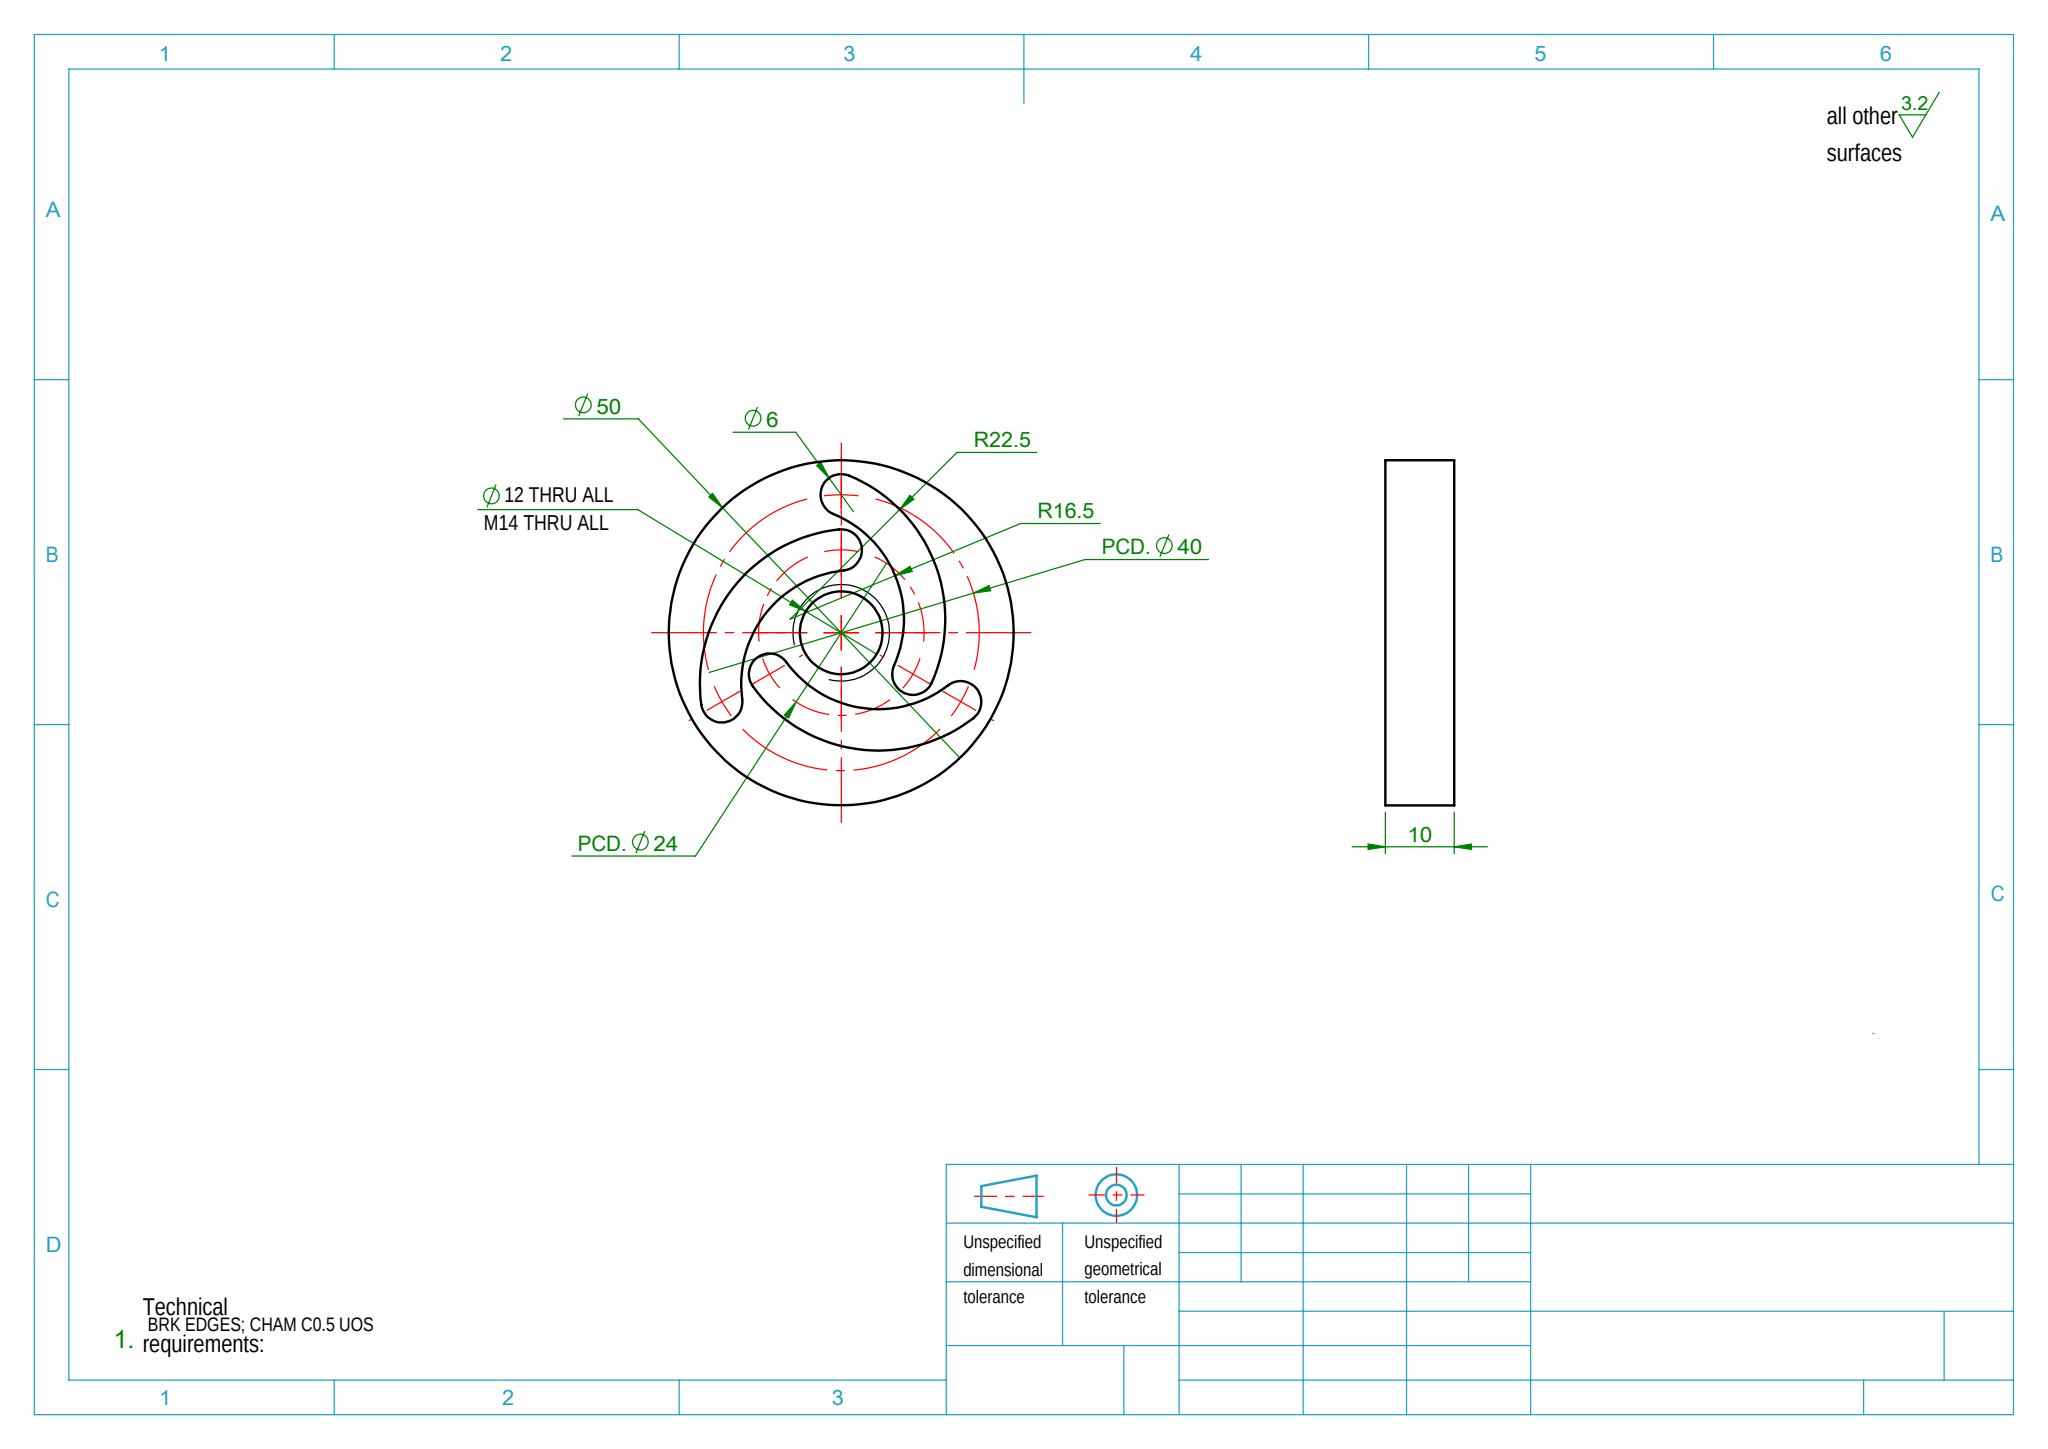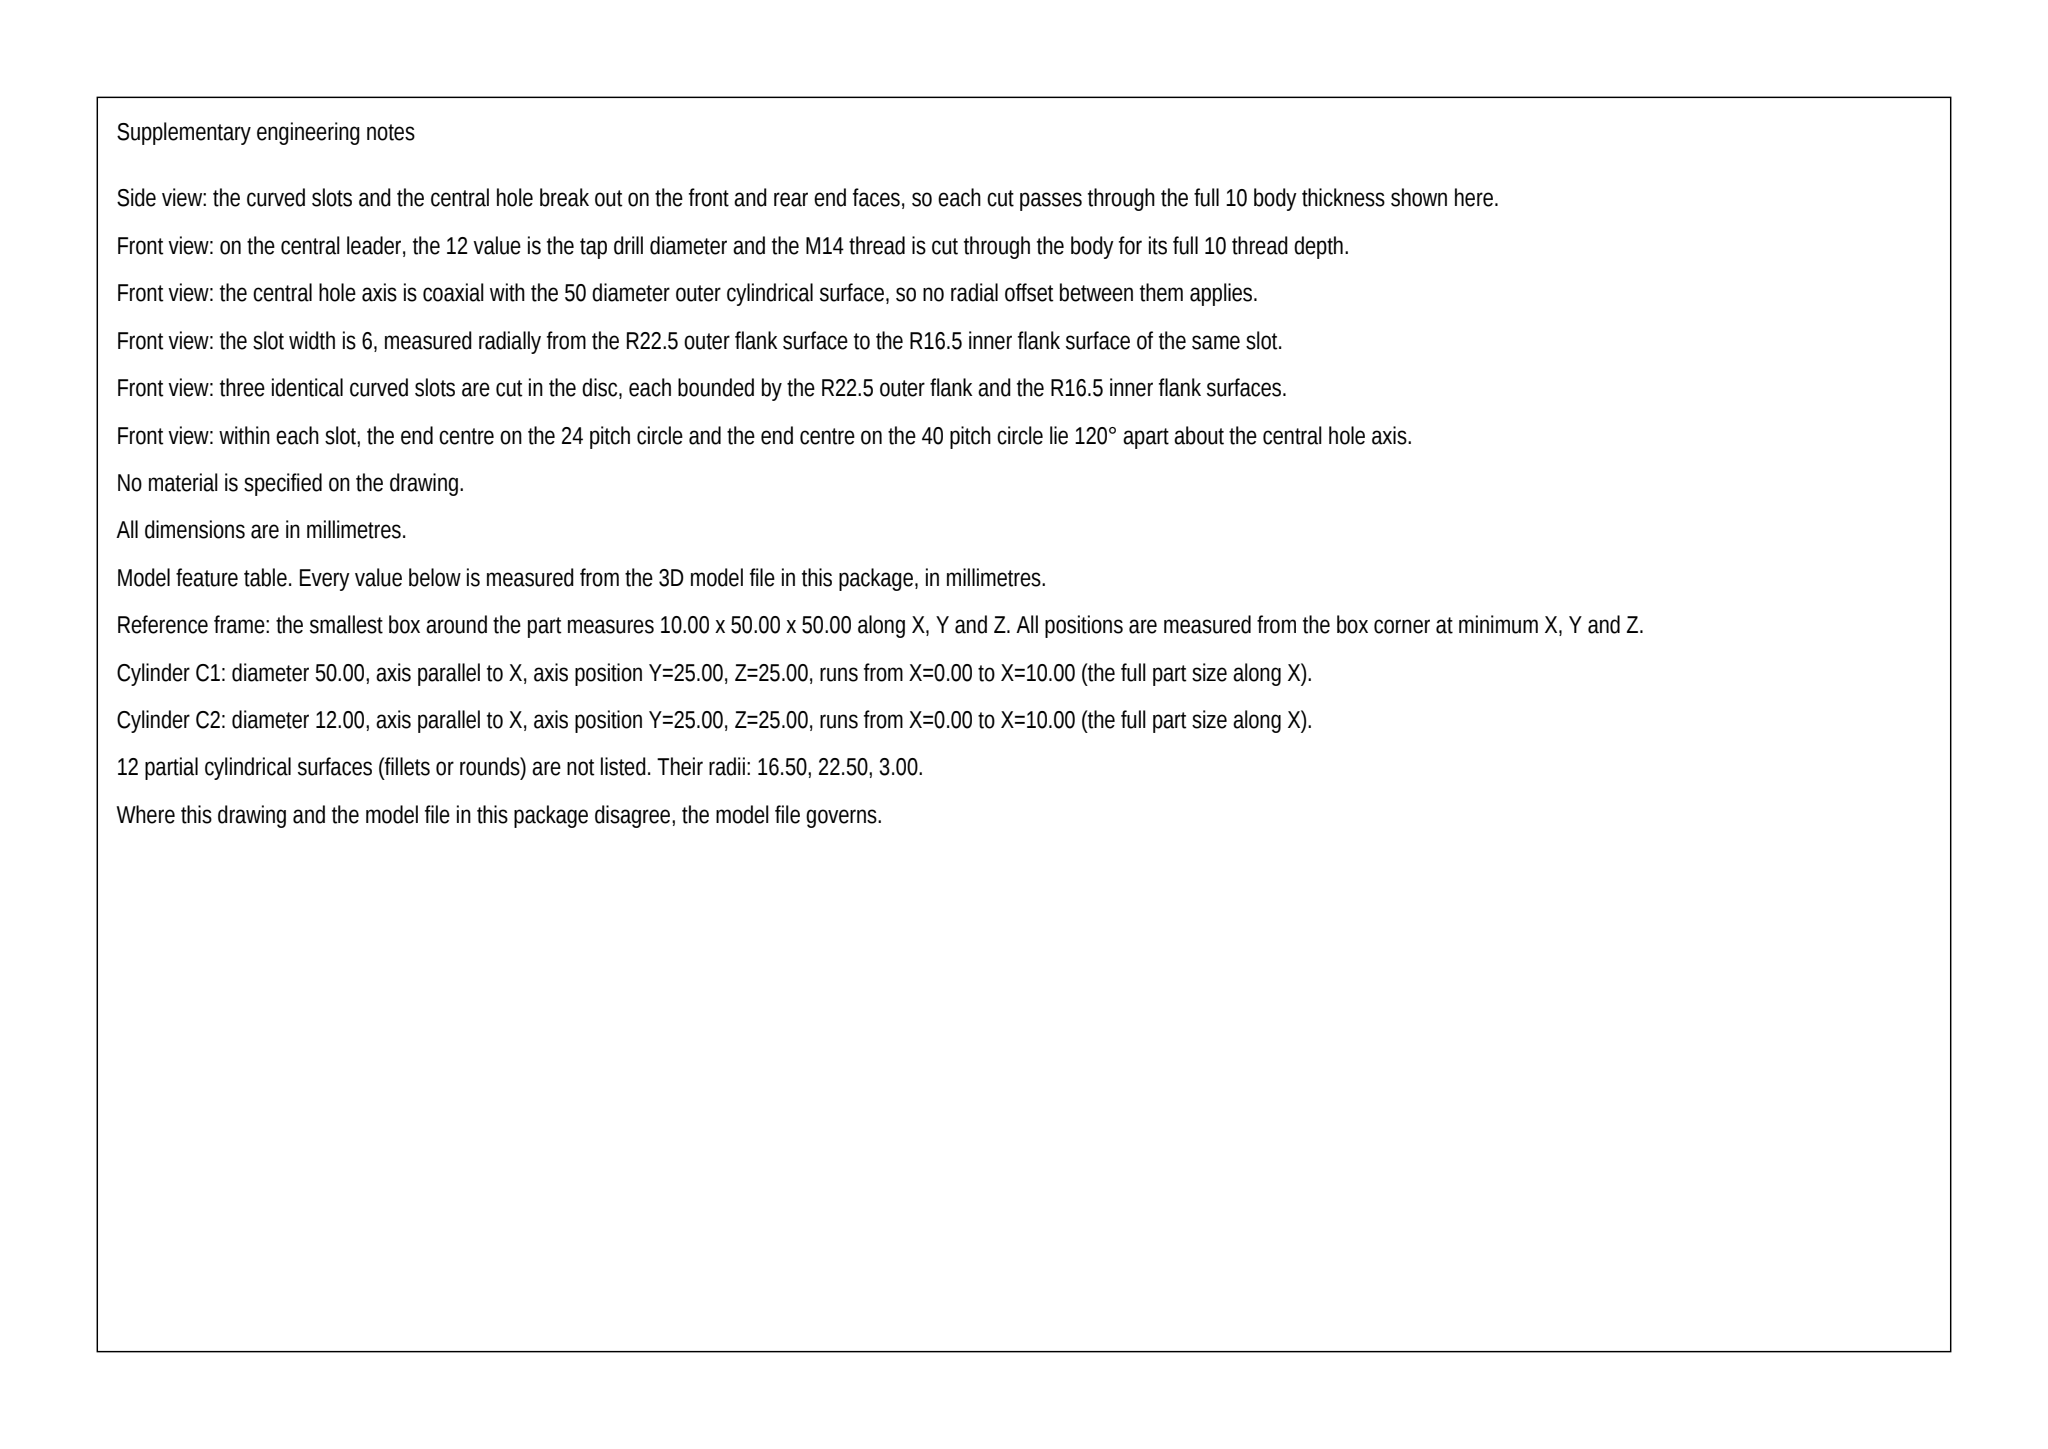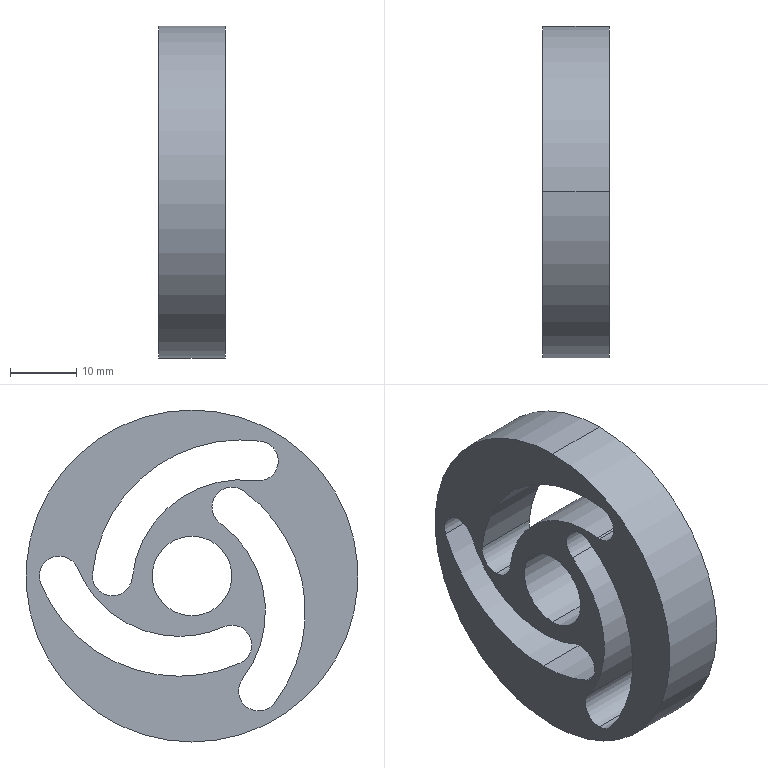Part | SolidWorks | mm | 1 solid | 23 faces | box 10 x 50 x 50 mm | volume 12034 mm3 | cylinder 21 | plane 2 | commonest cylinder face diameters 6 x9 33 x4 45 x4 12 x2 50 x2
Drawing notes:
3X SLOT ARC CTR: 7.67 FROM AXIS, 120° APART, R16.5/R22.5 | from the solid: R16.5/R22.5 arc centres at (17.6,23.0),(26.96,32.41),(30.43,19.6) vs part axis (25,25): offset 7.67, 120° apart
SLOT ENDS Ø6: PCD Ø24 END ON HORIZ CL, PCD Ø40 END 120° CCW | from the solid: Ø6 end-cap axes at r=12 (0°,120°,240°) and r=20 (0°,120°,240°) from axis (25,25); each slot links r=12 end to r=20 end 120° away, mean slot radius R19.5
3X CURVED SLOT THRU ALL (10) | from the solid: All Ø6/R16.5/R22.5 slot cylinders length 10 along x, between faces x=0 and x=10
build123d program:
from build123d import *

# Parameters (mm, degrees)
SKETCH1_R           = 25
BOSS_EXTRUDE1_DEPTH = 10
M14_TAPPED_HOLE1_D  = 12
CUT_EXTRUDE2_DEPTH  = 37.742
CIRPATTERN2_COUNT   = 3


with BuildPart() as part:
    # Sketch1 → Boss-Extrude1 (new body)
    with BuildSketch(Plane(origin=(0, 0, 0), x_dir=(0, 0, -1), z_dir=(1, 0, 0))):
        Circle(SKETCH1_R)
    extrude(amount=BOSS_EXTRUDE1_DEPTH)

    # M14 Tapped Hole1 (through all)
    with Locations(Plane(origin=(10, 0, 0), x_dir=(0, 0, -1), z_dir=(1, 0, 0))):
        with Locations((0, 0)):
            Hole(M14_TAPPED_HOLE1_D / 2)

    # Sketch7 → Cut-Extrude2 (cut, through all)
    with BuildSketch(Plane(origin=(10, 0, 0), x_dir=(0, 0, -1), z_dir=(1, 0, 0))):
        with BuildLine():
            ThreePointArc((-20.294, -10.401), (-16.92, -12.973), (-14.347, -9.599))
            ThreePointArc((-14.347, -9.599), (-10.959, 2.81), (0.3085, 9.016))
            ThreePointArc((0.3085, 9.016), (2.984, 12.308), (-0.3085, 14.984))
            ThreePointArc((-0.3085, 14.984), (-15.674, 6.522), (-20.294, -10.401))
        make_face()
    cut_extrude2 = extrude(amount=-CUT_EXTRUDE2_DEPTH, mode=Mode.SUBTRACT)

    # CirPattern2: Cut-Extrude2 ×3 about axis
    cirpattern2_axis = Axis((0, 0, 0), (1, 0, 0))
    for i in range(1, CIRPATTERN2_COUNT):
        add(cut_extrude2.rotate(cirpattern2_axis, i * 360 / CIRPATTERN2_COUNT), mode=Mode.SUBTRACT)


solid = part.part
STEP:
#1=CARTESIAN_POINT('',(0.,-10.,-20.321));
#2=VERTEX_POINT('',#1);
#3=CARTESIAN_POINT('',(0.,-7.625,-15.487));
#4=VERTEX_POINT('',#3);
#5=CARTESIAN_POINT('',(0.,-10.,-17.321));
#6=DIRECTION('',(1.,0.,0.));
#7=DIRECTION('',(0.,0.866,0.5));
#8=AXIS2_PLACEMENT_3D('',#5,#6,#7);
#9=CIRCLE('',#8,3.);
#10=EDGE_CURVE('',#2,#4,#9,.T.);
#11=ORIENTED_EDGE('',*,*,#10,.F.);
#12=CARTESIAN_POINT('',(10.,-10.,-20.321));
#13=VERTEX_POINT('',#12);
#14=CARTESIAN_POINT('',(0.,-10.,-20.321));
#15=DIRECTION('',(1.,0.,0.));
#16=VECTOR('',#15,1000.);
#17=LINE('',#14,#16);
#18=EDGE_CURVE('',#2,#13,#17,.T.);
#19=ORIENTED_EDGE('',*,*,#18,.T.);
#20=CARTESIAN_POINT('',(10.,-7.625,-15.487));
#21=VERTEX_POINT('',#20);
#22=CARTESIAN_POINT('',(10.,-10.,-17.321));
#23=DIRECTION('',(1.,0.,0.));
#24=DIRECTION('',(0.,0.866,0.5));
#25=AXIS2_PLACEMENT_3D('',#22,#23,#24);
#26=CIRCLE('',#25,3.);
#27=EDGE_CURVE('',#13,#21,#26,.T.);
#28=ORIENTED_EDGE('',*,*,#27,.T.);
#29=CARTESIAN_POINT('',(0.,-7.625,-15.487));
#30=DIRECTION('',(1.,0.,0.));
#31=VECTOR('',#30,1000.);
#32=LINE('',#29,#31);
#33=EDGE_CURVE('',#4,#21,#32,.T.);
#34=ORIENTED_EDGE('',*,*,#33,.F.);
#35=EDGE_LOOP('',(#11,#19,#28,#34));
#36=FACE_OUTER_BOUND('',#35,.T.);
#37=CARTESIAN_POINT('',(0.,-10.,-17.321));
#38=DIRECTION('',(1.,0.,0.));
#39=DIRECTION('',(0.,0.,-1.));
#40=AXIS2_PLACEMENT_3D('',#37,#38,#39);
#41=CYLINDRICAL_SURFACE('',#40,3.);
#42=ADVANCED_FACE('',(#36),#41,.F.);
#43=CARTESIAN_POINT('',(0.,1.962,-9.092));
#44=VERTEX_POINT('',#43);
#45=CARTESIAN_POINT('',(0.,-4.775,-7.654));
#46=VERTEX_POINT('',#45);
#47=CARTESIAN_POINT('',(0.,1.962,7.408));
#48=DIRECTION('',(-1.,0.,0.));
#49=DIRECTION('',(0.,-0.866,0.5));
#50=AXIS2_PLACEMENT_3D('',#47,#48,#49);
#51=CIRCLE('',#50,16.5);
#52=EDGE_CURVE('',#44,#46,#51,.T.);
#53=ORIENTED_EDGE('',*,*,#52,.F.);
#54=CARTESIAN_POINT('',(10.,1.962,-9.092));
#55=VERTEX_POINT('',#54);
#56=CARTESIAN_POINT('',(0.,1.962,-9.092));
#57=DIRECTION('',(1.,0.,0.));
#58=VECTOR('',#57,1000.);
#59=LINE('',#56,#58);
#60=EDGE_CURVE('',#44,#55,#59,.T.);
#61=ORIENTED_EDGE('',*,*,#60,.T.);
#62=CARTESIAN_POINT('',(10.,-4.775,-7.654));
#63=VERTEX_POINT('',#62);
#64=CARTESIAN_POINT('',(10.,1.962,7.408));
#65=DIRECTION('',(-1.,0.,0.));
#66=DIRECTION('',(0.,-0.866,0.5));
#67=AXIS2_PLACEMENT_3D('',#64,#65,#66);
#68=CIRCLE('',#67,16.5);
#69=EDGE_CURVE('',#55,#63,#68,.T.);
#70=ORIENTED_EDGE('',*,*,#69,.T.);
#71=CARTESIAN_POINT('',(0.,-4.775,-7.654));
#72=DIRECTION('',(1.,0.,0.));
#73=VECTOR('',#72,1000.);
#74=LINE('',#71,#73);
#75=EDGE_CURVE('',#46,#63,#74,.T.);
#76=ORIENTED_EDGE('',*,*,#75,.F.);
#77=EDGE_LOOP('',(#53,#61,#70,#76));
#78=FACE_OUTER_BOUND('',#77,.T.);
#79=CARTESIAN_POINT('',(0.,1.962,7.408));
#80=DIRECTION('',(1.,0.,0.));
#81=DIRECTION('',(0.,0.,-1.));
#82=AXIS2_PLACEMENT_3D('',#79,#80,#81);
#83=CYLINDRICAL_SURFACE('',#82,16.5);
#84=ADVANCED_FACE('',(#78),#83,.T.);
#85=CARTESIAN_POINT('',(0.,1.962,-15.092));
#86=VERTEX_POINT('',#85);
#87=CARTESIAN_POINT('',(0.,22.775,-1.14));
#88=VERTEX_POINT('',#87);
#89=CARTESIAN_POINT('',(0.,1.962,7.408));
#90=DIRECTION('',(1.,0.,0.));
#91=DIRECTION('',(0.,-0.866,0.5));
#92=AXIS2_PLACEMENT_3D('',#89,#90,#91);
#93=CIRCLE('',#92,22.5);
#94=EDGE_CURVE('',#86,#88,#93,.T.);
#95=ORIENTED_EDGE('',*,*,#94,.F.);
#96=CARTESIAN_POINT('',(10.,1.962,-15.092));
#97=VERTEX_POINT('',#96);
#98=CARTESIAN_POINT('',(0.,1.962,-15.092));
#99=DIRECTION('',(1.,0.,0.));
#100=VECTOR('',#99,1000.);
#101=LINE('',#98,#100);
#102=EDGE_CURVE('',#86,#97,#101,.T.);
#103=ORIENTED_EDGE('',*,*,#102,.T.);
#104=CARTESIAN_POINT('',(10.,22.775,-1.14));
#105=VERTEX_POINT('',#104);
#106=CARTESIAN_POINT('',(10.,1.962,7.408));
#107=DIRECTION('',(1.,0.,0.));
#108=DIRECTION('',(0.,-0.866,0.5));
#109=AXIS2_PLACEMENT_3D('',#106,#107,#108);
#110=CIRCLE('',#109,22.5);
#111=EDGE_CURVE('',#97,#105,#110,.T.);
#112=ORIENTED_EDGE('',*,*,#111,.T.);
#113=CARTESIAN_POINT('',(0.,22.775,-1.14));
#114=DIRECTION('',(1.,0.,0.));
#115=VECTOR('',#114,1000.);
#116=LINE('',#113,#115);
#117=EDGE_CURVE('',#88,#105,#116,.T.);
#118=ORIENTED_EDGE('',*,*,#117,.F.);
#119=EDGE_LOOP('',(#95,#103,#112,#118));
#120=FACE_OUTER_BOUND('',#119,.T.);
#121=CARTESIAN_POINT('',(0.,1.962,7.408));
#122=DIRECTION('',(1.,0.,0.));
#123=DIRECTION('',(0.,0.,-1.));
#124=AXIS2_PLACEMENT_3D('',#121,#122,#123);
#125=CYLINDRICAL_SURFACE('',#124,22.5);
#126=ADVANCED_FACE('',(#120),#125,.F.);
#127=CARTESIAN_POINT('',(0.,-10.,14.321));
#128=VERTEX_POINT('',#127);
#129=CARTESIAN_POINT('',(0.,-9.599,14.347));
#130=VERTEX_POINT('',#129);
#131=CARTESIAN_POINT('',(0.,-10.,17.321));
#132=DIRECTION('',(1.,0.,0.));
#133=DIRECTION('',(0.,0.,-1.));
#134=AXIS2_PLACEMENT_3D('',#131,#132,#133);
#135=CIRCLE('',#134,3.);
#136=EDGE_CURVE('',#128,#130,#135,.T.);
#137=ORIENTED_EDGE('',*,*,#136,.F.);
#138=CARTESIAN_POINT('',(10.,-10.,14.321));
#139=VERTEX_POINT('',#138);
#140=CARTESIAN_POINT('',(0.,-10.,14.321));
#141=DIRECTION('',(1.,0.,0.));
#142=VECTOR('',#141,1000.);
#143=LINE('',#140,#142);
#144=EDGE_CURVE('',#128,#139,#143,.T.);
#145=ORIENTED_EDGE('',*,*,#144,.T.);
#146=CARTESIAN_POINT('',(10.,-9.599,14.347));
#147=VERTEX_POINT('',#146);
#148=CARTESIAN_POINT('',(10.,-10.,17.321));
#149=DIRECTION('',(1.,0.,0.));
#150=DIRECTION('',(0.,0.,-1.));
#151=AXIS2_PLACEMENT_3D('',#148,#149,#150);
#152=CIRCLE('',#151,3.);
#153=EDGE_CURVE('',#139,#147,#152,.T.);
#154=ORIENTED_EDGE('',*,*,#153,.T.);
#155=CARTESIAN_POINT('',(0.,-9.599,14.347));
#156=DIRECTION('',(1.,0.,0.));
#157=VECTOR('',#156,1000.);
#158=LINE('',#155,#157);
#159=EDGE_CURVE('',#130,#147,#158,.T.);
#160=ORIENTED_EDGE('',*,*,#159,.F.);
#161=EDGE_LOOP('',(#137,#145,#154,#160));
#162=FACE_OUTER_BOUND('',#161,.T.);
#163=CARTESIAN_POINT('',(0.,-10.,17.321));
#164=DIRECTION('',(1.,0.,0.));
#165=DIRECTION('',(0.,0.,-1.));
#166=AXIS2_PLACEMENT_3D('',#163,#164,#165);
#167=CYLINDRICAL_SURFACE('',#166,3.);
#168=ADVANCED_FACE('',(#162),#167,.F.);
#169=CARTESIAN_POINT('',(0.,12.,-3.));
#170=VERTEX_POINT('',#169);
#171=CARTESIAN_POINT('',(0.,14.984,0.3085));
#172=VERTEX_POINT('',#171);
#173=CARTESIAN_POINT('',(0.,12.,0.));
#174=DIRECTION('',(1.,0.,0.));
#175=DIRECTION('',(0.,0.,-1.));
#176=AXIS2_PLACEMENT_3D('',#173,#174,#175);
#177=CIRCLE('',#176,3.);
#178=EDGE_CURVE('',#170,#172,#177,.T.);
#179=ORIENTED_EDGE('',*,*,#178,.F.);
#180=CARTESIAN_POINT('',(10.,12.,-3.));
#181=VERTEX_POINT('',#180);
#182=CARTESIAN_POINT('',(0.,12.,-3.));
#183=DIRECTION('',(1.,0.,0.));
#184=VECTOR('',#183,1000.);
#185=LINE('',#182,#184);
#186=EDGE_CURVE('',#170,#181,#185,.T.);
#187=ORIENTED_EDGE('',*,*,#186,.T.);
#188=CARTESIAN_POINT('',(10.,14.984,0.3085));
#189=VERTEX_POINT('',#188);
#190=CARTESIAN_POINT('',(10.,12.,0.));
#191=DIRECTION('',(1.,0.,0.));
#192=DIRECTION('',(0.,0.,-1.));
#193=AXIS2_PLACEMENT_3D('',#190,#191,#192);
#194=CIRCLE('',#193,3.);
#195=EDGE_CURVE('',#181,#189,#194,.T.);
#196=ORIENTED_EDGE('',*,*,#195,.T.);
#197=CARTESIAN_POINT('',(0.,14.984,0.3085));
#198=DIRECTION('',(1.,0.,0.));
#199=VECTOR('',#198,1000.);
#200=LINE('',#197,#199);
#201=EDGE_CURVE('',#172,#189,#200,.T.);
#202=ORIENTED_EDGE('',*,*,#201,.F.);
#203=EDGE_LOOP('',(#179,#187,#196,#202));
#204=FACE_OUTER_BOUND('',#203,.T.);
#205=CARTESIAN_POINT('',(0.,12.,0.));
#206=DIRECTION('',(1.,0.,0.));
#207=DIRECTION('',(0.,0.,-1.));
#208=AXIS2_PLACEMENT_3D('',#205,#206,#207);
#209=CYLINDRICAL_SURFACE('',#208,3.);
#210=ADVANCED_FACE('',(#204),#209,.F.);
#211=CARTESIAN_POINT('',(0.,0.,6.));
#212=VERTEX_POINT('',#211);
#213=CARTESIAN_POINT('',(0.,0.,-6.));
#214=VERTEX_POINT('',#213);
#215=CARTESIAN_POINT('',(0.,0.,0.));
#216=DIRECTION('',(1.,0.,0.));
#217=DIRECTION('',(0.,0.,-1.));
#218=AXIS2_PLACEMENT_3D('',#215,#216,#217);
#219=CIRCLE('',#218,6.);
#220=EDGE_CURVE('',#212,#214,#219,.T.);
#221=ORIENTED_EDGE('',*,*,#220,.F.);
#222=CARTESIAN_POINT('',(10.,0.,6.));
#223=VERTEX_POINT('',#222);
#224=CARTESIAN_POINT('',(10.,0.,6.));
#225=DIRECTION('',(1.,0.,0.));
#226=VECTOR('',#225,1000.);
#227=LINE('',#224,#226);
#228=EDGE_CURVE('',#212,#223,#227,.T.);
#229=ORIENTED_EDGE('',*,*,#228,.T.);
#230=CARTESIAN_POINT('',(10.,0.,-6.));
#231=VERTEX_POINT('',#230);
#232=CARTESIAN_POINT('',(10.,0.,0.));
#233=DIRECTION('',(1.,0.,0.));
#234=DIRECTION('',(0.,0.,-1.));
#235=AXIS2_PLACEMENT_3D('',#232,#233,#234);
#236=CIRCLE('',#235,6.);
#237=EDGE_CURVE('',#223,#231,#236,.T.);
#238=ORIENTED_EDGE('',*,*,#237,.T.);
#239=CARTESIAN_POINT('',(10.,0.,-6.));
#240=DIRECTION('',(1.,0.,0.));
#241=VECTOR('',#240,1000.);
#242=LINE('',#239,#241);
#243=EDGE_CURVE('',#214,#231,#242,.T.);
#244=ORIENTED_EDGE('',*,*,#243,.F.);
#245=EDGE_LOOP('',(#221,#229,#238,#244));
#246=FACE_OUTER_BOUND('',#245,.T.);
#247=CARTESIAN_POINT('',(10.,0.,0.));
#248=DIRECTION('',(1.,0.,0.));
#249=DIRECTION('',(0.,0.,-1.));
#250=AXIS2_PLACEMENT_3D('',#247,#248,#249);
#251=CYLINDRICAL_SURFACE('',#250,6.);
#252=ADVANCED_FACE('',(#246),#251,.F.);
#253=CARTESIAN_POINT('',(10.,0.,-25.));
#254=VERTEX_POINT('',#253);
#255=CARTESIAN_POINT('',(10.,0.,25.));
#256=VERTEX_POINT('',#255);
#257=CARTESIAN_POINT('',(10.,0.,0.));
#258=DIRECTION('',(1.,0.,0.));
#259=DIRECTION('',(0.,0.,-1.));
#260=AXIS2_PLACEMENT_3D('',#257,#258,#259);
#261=CIRCLE('',#260,25.);
#262=EDGE_CURVE('',#254,#256,#261,.T.);
#263=ORIENTED_EDGE('',*,*,#262,.F.);
#264=CARTESIAN_POINT('',(0.,0.,-25.));
#265=VERTEX_POINT('',#264);
#266=CARTESIAN_POINT('',(10.,0.,-25.));
#267=DIRECTION('',(-1.,0.,0.));
#268=VECTOR('',#267,1000.);
#269=LINE('',#266,#268);
#270=EDGE_CURVE('',#254,#265,#269,.T.);
#271=ORIENTED_EDGE('',*,*,#270,.T.);
#272=CARTESIAN_POINT('',(0.,0.,25.));
#273=VERTEX_POINT('',#272);
#274=CARTESIAN_POINT('',(0.,0.,0.));
#275=DIRECTION('',(1.,0.,0.));
#276=DIRECTION('',(0.,0.,-1.));
#277=AXIS2_PLACEMENT_3D('',#274,#275,#276);
#278=CIRCLE('',#277,25.);
#279=EDGE_CURVE('',#265,#273,#278,.T.);
#280=ORIENTED_EDGE('',*,*,#279,.T.);
#281=CARTESIAN_POINT('',(10.,0.,25.));
#282=DIRECTION('',(-1.,0.,0.));
#283=VECTOR('',#282,1000.);
#284=LINE('',#281,#283);
#285=EDGE_CURVE('',#256,#273,#284,.T.);
#286=ORIENTED_EDGE('',*,*,#285,.F.);
#287=EDGE_LOOP('',(#263,#271,#280,#286));
#288=FACE_OUTER_BOUND('',#287,.T.);
#289=CARTESIAN_POINT('',(10.,0.,0.));
#290=DIRECTION('',(-1.,0.,0.));
#291=DIRECTION('',(0.,0.,1.));
#292=AXIS2_PLACEMENT_3D('',#289,#290,#291);
#293=CYLINDRICAL_SURFACE('',#292,25.);
#294=ADVANCED_FACE('',(#288),#293,.T.);
#295=ORIENTED_EDGE('',*,*,#270,.F.);
#296=CARTESIAN_POINT('',(10.,0.,0.));
#297=DIRECTION('',(1.,0.,0.));
#298=DIRECTION('',(0.,0.,-1.));
#299=AXIS2_PLACEMENT_3D('',#296,#297,#298);
#300=CIRCLE('',#299,25.);
#301=EDGE_CURVE('',#256,#254,#300,.T.);
#302=ORIENTED_EDGE('',*,*,#301,.F.);
#303=ORIENTED_EDGE('',*,*,#285,.T.);
#304=CARTESIAN_POINT('',(0.,0.,0.));
#305=DIRECTION('',(1.,0.,0.));
#306=DIRECTION('',(0.,0.,-1.));
#307=AXIS2_PLACEMENT_3D('',#304,#305,#306);
#308=CIRCLE('',#307,25.);
#309=EDGE_CURVE('',#273,#265,#308,.T.);
#310=ORIENTED_EDGE('',*,*,#309,.T.);
#311=EDGE_LOOP('',(#295,#302,#303,#310));
#312=FACE_OUTER_BOUND('',#311,.T.);
#313=CARTESIAN_POINT('',(10.,0.,0.));
#314=DIRECTION('',(-1.,0.,0.));
#315=DIRECTION('',(0.,0.,1.));
#316=AXIS2_PLACEMENT_3D('',#313,#314,#315);
#317=CYLINDRICAL_SURFACE('',#316,25.);
#318=ADVANCED_FACE('',(#312),#317,.T.);
#319=CARTESIAN_POINT('',(10.,-7.759,12.822));
#320=VERTEX_POINT('',#319);
#321=CARTESIAN_POINT('',(10.,-12.375,-19.154));
#322=VERTEX_POINT('',#321);
#323=CARTESIAN_POINT('',(10.,5.435,-5.403));
#324=DIRECTION('',(1.,0.,0.));
#325=DIRECTION('',(0.,0.866,0.5));
#326=AXIS2_PLACEMENT_3D('',#323,#324,#325);
#327=CIRCLE('',#326,22.5);
#328=EDGE_CURVE('',#320,#322,#327,.T.);
#329=ORIENTED_EDGE('',*,*,#328,.F.);
#330=CARTESIAN_POINT('',(10.,-4.241,7.962));
#331=VERTEX_POINT('',#330);
#332=CARTESIAN_POINT('',(10.,-6.,10.392));
#333=DIRECTION('',(1.,0.,0.));
#334=DIRECTION('',(0.,0.866,0.5));
#335=AXIS2_PLACEMENT_3D('',#332,#333,#334);
#336=CIRCLE('',#335,3.);
#337=EDGE_CURVE('',#331,#320,#336,.T.);
#338=ORIENTED_EDGE('',*,*,#337,.F.);
#339=CARTESIAN_POINT('',(10.,5.435,-5.403));
#340=DIRECTION('',(-1.,0.,0.));
#341=DIRECTION('',(0.,0.866,0.5));
#342=AXIS2_PLACEMENT_3D('',#339,#340,#341);
#343=CIRCLE('',#342,16.5);
#344=EDGE_CURVE('',#21,#331,#343,.T.);
#345=ORIENTED_EDGE('',*,*,#344,.F.);
#346=ORIENTED_EDGE('',*,*,#27,.F.);
#347=CARTESIAN_POINT('',(10.,-10.,-17.321));
#348=DIRECTION('',(1.,0.,0.));
#349=DIRECTION('',(0.,0.866,0.5));
#350=AXIS2_PLACEMENT_3D('',#347,#348,#349);
#351=CIRCLE('',#350,3.);
#352=EDGE_CURVE('',#322,#13,#351,.T.);
#353=ORIENTED_EDGE('',*,*,#352,.F.);
#354=EDGE_LOOP('',(#329,#338,#345,#346,#353));
#355=FACE_BOUND('',#354,.T.);
#356=CARTESIAN_POINT('',(10.,-7.225,-13.131));
#357=VERTEX_POINT('',#356);
#358=CARTESIAN_POINT('',(10.,1.962,7.408));
#359=DIRECTION('',(1.,0.,0.));
#360=DIRECTION('',(0.,-0.866,0.5));
#361=AXIS2_PLACEMENT_3D('',#358,#359,#360);
#362=CIRCLE('',#361,22.5);
#363=EDGE_CURVE('',#357,#97,#362,.T.);
#364=ORIENTED_EDGE('',*,*,#363,.F.);
#365=CARTESIAN_POINT('',(10.,-6.,-10.392));
#366=DIRECTION('',(1.,0.,0.));
#367=DIRECTION('',(0.,-0.866,0.5));
#368=AXIS2_PLACEMENT_3D('',#365,#366,#367);
#369=CIRCLE('',#368,3.);
#370=EDGE_CURVE('',#63,#357,#369,.T.);
#371=ORIENTED_EDGE('',*,*,#370,.F.);
#372=ORIENTED_EDGE('',*,*,#69,.F.);
#373=CARTESIAN_POINT('',(10.,17.225,1.14));
#374=VERTEX_POINT('',#373);
#375=CARTESIAN_POINT('',(10.,1.962,7.408));
#376=DIRECTION('',(-1.,0.,0.));
#377=DIRECTION('',(0.,-0.866,0.5));
#378=AXIS2_PLACEMENT_3D('',#375,#376,#377);
#379=CIRCLE('',#378,16.5);
#380=EDGE_CURVE('',#374,#55,#379,.T.);
#381=ORIENTED_EDGE('',*,*,#380,.F.);
#382=CARTESIAN_POINT('',(10.,20.,0.));
#383=DIRECTION('',(1.,0.,0.));
#384=DIRECTION('',(0.,-0.866,0.5));
#385=AXIS2_PLACEMENT_3D('',#382,#383,#384);
#386=CIRCLE('',#385,3.);
#387=EDGE_CURVE('',#105,#374,#386,.T.);
#388=ORIENTED_EDGE('',*,*,#387,.F.);
#389=ORIENTED_EDGE('',*,*,#111,.F.);
#390=EDGE_LOOP('',(#364,#371,#372,#381,#388,#389));
#391=FACE_BOUND('',#390,.T.);
#392=CARTESIAN_POINT('',(10.,-10.401,20.294));
#393=VERTEX_POINT('',#392);
#394=CARTESIAN_POINT('',(10.,-7.397,-2.005));
#395=DIRECTION('',(1.,0.,0.));
#396=DIRECTION('',(0.,0.,-1.));
#397=AXIS2_PLACEMENT_3D('',#394,#395,#396);
#398=CIRCLE('',#397,22.5);
#399=EDGE_CURVE('',#189,#393,#398,.T.);
#400=ORIENTED_EDGE('',*,*,#399,.F.);
#401=ORIENTED_EDGE('',*,*,#195,.F.);
#402=CARTESIAN_POINT('',(10.,9.016,-0.3085));
#403=VERTEX_POINT('',#402);
#404=CARTESIAN_POINT('',(10.,12.,0.));
#405=DIRECTION('',(1.,0.,0.));
#406=DIRECTION('',(0.,0.,-1.));
#407=AXIS2_PLACEMENT_3D('',#404,#405,#406);
#408=CIRCLE('',#407,3.);
#409=EDGE_CURVE('',#403,#181,#408,.T.);
#410=ORIENTED_EDGE('',*,*,#409,.F.);
#411=CARTESIAN_POINT('',(10.,-7.397,-2.005));
#412=DIRECTION('',(-1.,0.,0.));
#413=DIRECTION('',(0.,0.,-1.));
#414=AXIS2_PLACEMENT_3D('',#411,#412,#413);
#415=CIRCLE('',#414,16.5);
#416=EDGE_CURVE('',#147,#403,#415,.T.);
#417=ORIENTED_EDGE('',*,*,#416,.F.);
#418=ORIENTED_EDGE('',*,*,#153,.F.);
#419=CARTESIAN_POINT('',(10.,-10.,17.321));
#420=DIRECTION('',(1.,0.,0.));
#421=DIRECTION('',(0.,0.,-1.));
#422=AXIS2_PLACEMENT_3D('',#419,#420,#421);
#423=CIRCLE('',#422,3.);
#424=EDGE_CURVE('',#393,#139,#423,.T.);
#425=ORIENTED_EDGE('',*,*,#424,.F.);
#426=EDGE_LOOP('',(#400,#401,#410,#417,#418,#425));
#427=FACE_BOUND('',#426,.T.);
#428=CARTESIAN_POINT('',(10.,0.,0.));
#429=DIRECTION('',(1.,0.,0.));
#430=DIRECTION('',(0.,0.,-1.));
#431=AXIS2_PLACEMENT_3D('',#428,#429,#430);
#432=CIRCLE('',#431,6.);
#433=EDGE_CURVE('',#231,#223,#432,.T.);
#434=ORIENTED_EDGE('',*,*,#433,.F.);
#435=ORIENTED_EDGE('',*,*,#237,.F.);
#436=EDGE_LOOP('',(#434,#435));
#437=FACE_BOUND('',#436,.T.);
#438=ORIENTED_EDGE('',*,*,#301,.T.);
#439=ORIENTED_EDGE('',*,*,#262,.T.);
#440=EDGE_LOOP('',(#438,#439));
#441=FACE_OUTER_BOUND('',#440,.T.);
#442=CARTESIAN_POINT('',(10.,0.,0.));
#443=DIRECTION('',(1.,0.,0.));
#444=DIRECTION('',(0.,0.,-1.));
#445=AXIS2_PLACEMENT_3D('',#442,#443,#444);
#446=PLANE('',#445);
#447=ADVANCED_FACE('',(#355,#391,#427,#437,#441),#446,.T.);
#448=CARTESIAN_POINT('',(0.,-4.241,7.962));
#449=VERTEX_POINT('',#448);
#450=CARTESIAN_POINT('',(0.,-7.759,12.822));
#451=VERTEX_POINT('',#450);
#452=CARTESIAN_POINT('',(0.,-6.,10.392));
#453=DIRECTION('',(1.,0.,0.));
#454=DIRECTION('',(0.,0.866,0.5));
#455=AXIS2_PLACEMENT_3D('',#452,#453,#454);
#456=CIRCLE('',#455,3.);
#457=EDGE_CURVE('',#449,#451,#456,.T.);
#458=ORIENTED_EDGE('',*,*,#457,.T.);
#459=CARTESIAN_POINT('',(0.,-12.375,-19.154));
#460=VERTEX_POINT('',#459);
#461=CARTESIAN_POINT('',(0.,5.435,-5.403));
#462=DIRECTION('',(1.,0.,0.));
#463=DIRECTION('',(0.,0.866,0.5));
#464=AXIS2_PLACEMENT_3D('',#461,#462,#463);
#465=CIRCLE('',#464,22.5);
#466=EDGE_CURVE('',#451,#460,#465,.T.);
#467=ORIENTED_EDGE('',*,*,#466,.T.);
#468=CARTESIAN_POINT('',(0.,-10.,-17.321));
#469=DIRECTION('',(1.,0.,0.));
#470=DIRECTION('',(0.,0.866,0.5));
#471=AXIS2_PLACEMENT_3D('',#468,#469,#470);
#472=CIRCLE('',#471,3.);
#473=EDGE_CURVE('',#460,#2,#472,.T.);
#474=ORIENTED_EDGE('',*,*,#473,.T.);
#475=ORIENTED_EDGE('',*,*,#10,.T.);
#476=CARTESIAN_POINT('',(0.,5.435,-5.403));
#477=DIRECTION('',(-1.,0.,0.));
#478=DIRECTION('',(0.,0.866,0.5));
#479=AXIS2_PLACEMENT_3D('',#476,#477,#478);
#480=CIRCLE('',#479,16.5);
#481=EDGE_CURVE('',#4,#449,#480,.T.);
#482=ORIENTED_EDGE('',*,*,#481,.T.);
#483=EDGE_LOOP('',(#458,#467,#474,#475,#482));
#484=FACE_BOUND('',#483,.T.);
#485=CARTESIAN_POINT('',(0.,-7.225,-13.131));
#486=VERTEX_POINT('',#485);
#487=CARTESIAN_POINT('',(0.,-6.,-10.392));
#488=DIRECTION('',(1.,0.,0.));
#489=DIRECTION('',(0.,-0.866,0.5));
#490=AXIS2_PLACEMENT_3D('',#487,#488,#489);
#491=CIRCLE('',#490,3.);
#492=EDGE_CURVE('',#46,#486,#491,.T.);
#493=ORIENTED_EDGE('',*,*,#492,.T.);
#494=CARTESIAN_POINT('',(0.,1.962,7.408));
#495=DIRECTION('',(1.,0.,0.));
#496=DIRECTION('',(0.,-0.866,0.5));
#497=AXIS2_PLACEMENT_3D('',#494,#495,#496);
#498=CIRCLE('',#497,22.5);
#499=EDGE_CURVE('',#486,#86,#498,.T.);
#500=ORIENTED_EDGE('',*,*,#499,.T.);
#501=ORIENTED_EDGE('',*,*,#94,.T.);
#502=CARTESIAN_POINT('',(0.,17.225,1.14));
#503=VERTEX_POINT('',#502);
#504=CARTESIAN_POINT('',(0.,20.,0.));
#505=DIRECTION('',(1.,0.,0.));
#506=DIRECTION('',(0.,-0.866,0.5));
#507=AXIS2_PLACEMENT_3D('',#504,#505,#506);
#508=CIRCLE('',#507,3.);
#509=EDGE_CURVE('',#88,#503,#508,.T.);
#510=ORIENTED_EDGE('',*,*,#509,.T.);
#511=CARTESIAN_POINT('',(0.,1.962,7.408));
#512=DIRECTION('',(-1.,0.,0.));
#513=DIRECTION('',(0.,-0.866,0.5));
#514=AXIS2_PLACEMENT_3D('',#511,#512,#513);
#515=CIRCLE('',#514,16.5);
#516=EDGE_CURVE('',#503,#44,#515,.T.);
#517=ORIENTED_EDGE('',*,*,#516,.T.);
#518=ORIENTED_EDGE('',*,*,#52,.T.);
#519=EDGE_LOOP('',(#493,#500,#501,#510,#517,#518));
#520=FACE_BOUND('',#519,.T.);
#521=CARTESIAN_POINT('',(0.,9.016,-0.3085));
#522=VERTEX_POINT('',#521);
#523=CARTESIAN_POINT('',(0.,12.,0.));
#524=DIRECTION('',(1.,0.,0.));
#525=DIRECTION('',(0.,0.,-1.));
#526=AXIS2_PLACEMENT_3D('',#523,#524,#525);
#527=CIRCLE('',#526,3.);
#528=EDGE_CURVE('',#522,#170,#527,.T.);
#529=ORIENTED_EDGE('',*,*,#528,.T.);
#530=ORIENTED_EDGE('',*,*,#178,.T.);
#531=CARTESIAN_POINT('',(0.,-10.401,20.294));
#532=VERTEX_POINT('',#531);
#533=CARTESIAN_POINT('',(0.,-7.397,-2.005));
#534=DIRECTION('',(1.,0.,0.));
#535=DIRECTION('',(0.,0.,-1.));
#536=AXIS2_PLACEMENT_3D('',#533,#534,#535);
#537=CIRCLE('',#536,22.5);
#538=EDGE_CURVE('',#172,#532,#537,.T.);
#539=ORIENTED_EDGE('',*,*,#538,.T.);
#540=CARTESIAN_POINT('',(0.,-10.,17.321));
#541=DIRECTION('',(1.,0.,0.));
#542=DIRECTION('',(0.,0.,-1.));
#543=AXIS2_PLACEMENT_3D('',#540,#541,#542);
#544=CIRCLE('',#543,3.);
#545=EDGE_CURVE('',#532,#128,#544,.T.);
#546=ORIENTED_EDGE('',*,*,#545,.T.);
#547=ORIENTED_EDGE('',*,*,#136,.T.);
#548=CARTESIAN_POINT('',(0.,-7.397,-2.005));
#549=DIRECTION('',(-1.,0.,0.));
#550=DIRECTION('',(0.,0.,-1.));
#551=AXIS2_PLACEMENT_3D('',#548,#549,#550);
#552=CIRCLE('',#551,16.5);
#553=EDGE_CURVE('',#130,#522,#552,.T.);
#554=ORIENTED_EDGE('',*,*,#553,.T.);
#555=EDGE_LOOP('',(#529,#530,#539,#546,#547,#554));
#556=FACE_BOUND('',#555,.T.);
#557=CARTESIAN_POINT('',(0.,0.,0.));
#558=DIRECTION('',(1.,0.,0.));
#559=DIRECTION('',(0.,0.,-1.));
#560=AXIS2_PLACEMENT_3D('',#557,#558,#559);
#561=CIRCLE('',#560,6.);
#562=EDGE_CURVE('',#214,#212,#561,.T.);
#563=ORIENTED_EDGE('',*,*,#562,.T.);
#564=ORIENTED_EDGE('',*,*,#220,.T.);
#565=EDGE_LOOP('',(#563,#564));
#566=FACE_BOUND('',#565,.T.);
#567=ORIENTED_EDGE('',*,*,#309,.F.);
#568=ORIENTED_EDGE('',*,*,#279,.F.);
#569=EDGE_LOOP('',(#567,#568));
#570=FACE_OUTER_BOUND('',#569,.T.);
#571=CARTESIAN_POINT('',(0.,0.,0.));
#572=DIRECTION('',(1.,0.,0.));
#573=DIRECTION('',(0.,0.,-1.));
#574=AXIS2_PLACEMENT_3D('',#571,#572,#573);
#575=PLANE('',#574);
#576=ADVANCED_FACE('',(#484,#520,#556,#566,#570),#575,.F.);
#577=ORIENTED_EDGE('',*,*,#228,.F.);
#578=ORIENTED_EDGE('',*,*,#562,.F.);
#579=ORIENTED_EDGE('',*,*,#243,.T.);
#580=ORIENTED_EDGE('',*,*,#433,.T.);
#581=EDGE_LOOP('',(#577,#578,#579,#580));
#582=FACE_OUTER_BOUND('',#581,.T.);
#583=CARTESIAN_POINT('',(10.,0.,0.));
#584=DIRECTION('',(1.,0.,0.));
#585=DIRECTION('',(0.,0.,-1.));
#586=AXIS2_PLACEMENT_3D('',#583,#584,#585);
#587=CYLINDRICAL_SURFACE('',#586,6.);
#588=ADVANCED_FACE('',(#582),#587,.F.);
#589=ORIENTED_EDGE('',*,*,#399,.T.);
#590=CARTESIAN_POINT('',(0.,-10.401,20.294));
#591=DIRECTION('',(1.,0.,0.));
#592=VECTOR('',#591,1000.);
#593=LINE('',#590,#592);
#594=EDGE_CURVE('',#532,#393,#593,.T.);
#595=ORIENTED_EDGE('',*,*,#594,.F.);
#596=ORIENTED_EDGE('',*,*,#538,.F.);
#597=ORIENTED_EDGE('',*,*,#201,.T.);
#598=EDGE_LOOP('',(#589,#595,#596,#597));
#599=FACE_OUTER_BOUND('',#598,.T.);
#600=CARTESIAN_POINT('',(0.,-7.397,-2.005));
#601=DIRECTION('',(1.,0.,0.));
#602=DIRECTION('',(0.,0.,-1.));
#603=AXIS2_PLACEMENT_3D('',#600,#601,#602);
#604=CYLINDRICAL_SURFACE('',#603,22.5);
#605=ADVANCED_FACE('',(#599),#604,.F.);
#606=ORIENTED_EDGE('',*,*,#186,.F.);
#607=ORIENTED_EDGE('',*,*,#528,.F.);
#608=CARTESIAN_POINT('',(0.,9.016,-0.3085));
#609=DIRECTION('',(1.,0.,0.));
#610=VECTOR('',#609,1000.);
#611=LINE('',#608,#610);
#612=EDGE_CURVE('',#522,#403,#611,.T.);
#613=ORIENTED_EDGE('',*,*,#612,.T.);
#614=ORIENTED_EDGE('',*,*,#409,.T.);
#615=EDGE_LOOP('',(#606,#607,#613,#614));
#616=FACE_OUTER_BOUND('',#615,.T.);
#617=CARTESIAN_POINT('',(0.,12.,0.));
#618=DIRECTION('',(1.,0.,0.));
#619=DIRECTION('',(0.,0.,-1.));
#620=AXIS2_PLACEMENT_3D('',#617,#618,#619);
#621=CYLINDRICAL_SURFACE('',#620,3.);
#622=ADVANCED_FACE('',(#616),#621,.F.);
#623=ORIENTED_EDGE('',*,*,#416,.T.);
#624=ORIENTED_EDGE('',*,*,#612,.F.);
#625=ORIENTED_EDGE('',*,*,#553,.F.);
#626=ORIENTED_EDGE('',*,*,#159,.T.);
#627=EDGE_LOOP('',(#623,#624,#625,#626));
#628=FACE_OUTER_BOUND('',#627,.T.);
#629=CARTESIAN_POINT('',(0.,-7.397,-2.005));
#630=DIRECTION('',(1.,0.,0.));
#631=DIRECTION('',(0.,0.,-1.));
#632=AXIS2_PLACEMENT_3D('',#629,#630,#631);
#633=CYLINDRICAL_SURFACE('',#632,16.5);
#634=ADVANCED_FACE('',(#628),#633,.T.);
#635=ORIENTED_EDGE('',*,*,#144,.F.);
#636=ORIENTED_EDGE('',*,*,#545,.F.);
#637=ORIENTED_EDGE('',*,*,#594,.T.);
#638=ORIENTED_EDGE('',*,*,#424,.T.);
#639=EDGE_LOOP('',(#635,#636,#637,#638));
#640=FACE_OUTER_BOUND('',#639,.T.);
#641=CARTESIAN_POINT('',(0.,-10.,17.321));
#642=DIRECTION('',(1.,0.,0.));
#643=DIRECTION('',(0.,0.,-1.));
#644=AXIS2_PLACEMENT_3D('',#641,#642,#643);
#645=CYLINDRICAL_SURFACE('',#644,3.);
#646=ADVANCED_FACE('',(#640),#645,.F.);
#647=ORIENTED_EDGE('',*,*,#102,.F.);
#648=ORIENTED_EDGE('',*,*,#499,.F.);
#649=CARTESIAN_POINT('',(0.,-7.225,-13.131));
#650=DIRECTION('',(1.,0.,0.));
#651=VECTOR('',#650,1000.);
#652=LINE('',#649,#651);
#653=EDGE_CURVE('',#486,#357,#652,.T.);
#654=ORIENTED_EDGE('',*,*,#653,.T.);
#655=ORIENTED_EDGE('',*,*,#363,.T.);
#656=EDGE_LOOP('',(#647,#648,#654,#655));
#657=FACE_OUTER_BOUND('',#656,.T.);
#658=CARTESIAN_POINT('',(0.,1.962,7.408));
#659=DIRECTION('',(1.,0.,0.));
#660=DIRECTION('',(0.,0.,-1.));
#661=AXIS2_PLACEMENT_3D('',#658,#659,#660);
#662=CYLINDRICAL_SURFACE('',#661,22.5);
#663=ADVANCED_FACE('',(#657),#662,.F.);
#664=ORIENTED_EDGE('',*,*,#370,.T.);
#665=ORIENTED_EDGE('',*,*,#653,.F.);
#666=ORIENTED_EDGE('',*,*,#492,.F.);
#667=ORIENTED_EDGE('',*,*,#75,.T.);
#668=EDGE_LOOP('',(#664,#665,#666,#667));
#669=FACE_OUTER_BOUND('',#668,.T.);
#670=CARTESIAN_POINT('',(0.,-6.,-10.392));
#671=DIRECTION('',(1.,0.,0.));
#672=DIRECTION('',(0.,0.,-1.));
#673=AXIS2_PLACEMENT_3D('',#670,#671,#672);
#674=CYLINDRICAL_SURFACE('',#673,3.);
#675=ADVANCED_FACE('',(#669),#674,.F.);
#676=ORIENTED_EDGE('',*,*,#60,.F.);
#677=ORIENTED_EDGE('',*,*,#516,.F.);
#678=CARTESIAN_POINT('',(0.,17.225,1.14));
#679=DIRECTION('',(1.,0.,0.));
#680=VECTOR('',#679,1000.);
#681=LINE('',#678,#680);
#682=EDGE_CURVE('',#503,#374,#681,.T.);
#683=ORIENTED_EDGE('',*,*,#682,.T.);
#684=ORIENTED_EDGE('',*,*,#380,.T.);
#685=EDGE_LOOP('',(#676,#677,#683,#684));
#686=FACE_OUTER_BOUND('',#685,.T.);
#687=CARTESIAN_POINT('',(0.,1.962,7.408));
#688=DIRECTION('',(1.,0.,0.));
#689=DIRECTION('',(0.,0.,-1.));
#690=AXIS2_PLACEMENT_3D('',#687,#688,#689);
#691=CYLINDRICAL_SURFACE('',#690,16.5);
#692=ADVANCED_FACE('',(#686),#691,.T.);
#693=ORIENTED_EDGE('',*,*,#387,.T.);
#694=ORIENTED_EDGE('',*,*,#682,.F.);
#695=ORIENTED_EDGE('',*,*,#509,.F.);
#696=ORIENTED_EDGE('',*,*,#117,.T.);
#697=EDGE_LOOP('',(#693,#694,#695,#696));
#698=FACE_OUTER_BOUND('',#697,.T.);
#699=CARTESIAN_POINT('',(0.,20.,0.));
#700=DIRECTION('',(1.,0.,0.));
#701=DIRECTION('',(0.,0.,-1.));
#702=AXIS2_PLACEMENT_3D('',#699,#700,#701);
#703=CYLINDRICAL_SURFACE('',#702,3.);
#704=ADVANCED_FACE('',(#698),#703,.F.);
#705=ORIENTED_EDGE('',*,*,#328,.T.);
#706=CARTESIAN_POINT('',(0.,-12.375,-19.154));
#707=DIRECTION('',(1.,0.,0.));
#708=VECTOR('',#707,1000.);
#709=LINE('',#706,#708);
#710=EDGE_CURVE('',#460,#322,#709,.T.);
#711=ORIENTED_EDGE('',*,*,#710,.F.);
#712=ORIENTED_EDGE('',*,*,#466,.F.);
#713=CARTESIAN_POINT('',(0.,-7.759,12.822));
#714=DIRECTION('',(1.,0.,0.));
#715=VECTOR('',#714,1000.);
#716=LINE('',#713,#715);
#717=EDGE_CURVE('',#451,#320,#716,.T.);
#718=ORIENTED_EDGE('',*,*,#717,.T.);
#719=EDGE_LOOP('',(#705,#711,#712,#718));
#720=FACE_OUTER_BOUND('',#719,.T.);
#721=CARTESIAN_POINT('',(0.,5.435,-5.403));
#722=DIRECTION('',(1.,0.,0.));
#723=DIRECTION('',(0.,0.,-1.));
#724=AXIS2_PLACEMENT_3D('',#721,#722,#723);
#725=CYLINDRICAL_SURFACE('',#724,22.5);
#726=ADVANCED_FACE('',(#720),#725,.F.);
#727=ORIENTED_EDGE('',*,*,#337,.T.);
#728=ORIENTED_EDGE('',*,*,#717,.F.);
#729=ORIENTED_EDGE('',*,*,#457,.F.);
#730=CARTESIAN_POINT('',(0.,-4.241,7.962));
#731=DIRECTION('',(1.,0.,0.));
#732=VECTOR('',#731,1000.);
#733=LINE('',#730,#732);
#734=EDGE_CURVE('',#449,#331,#733,.T.);
#735=ORIENTED_EDGE('',*,*,#734,.T.);
#736=EDGE_LOOP('',(#727,#728,#729,#735));
#737=FACE_OUTER_BOUND('',#736,.T.);
#738=CARTESIAN_POINT('',(0.,-6.,10.392));
#739=DIRECTION('',(1.,0.,0.));
#740=DIRECTION('',(0.,0.,-1.));
#741=AXIS2_PLACEMENT_3D('',#738,#739,#740);
#742=CYLINDRICAL_SURFACE('',#741,3.);
#743=ADVANCED_FACE('',(#737),#742,.F.);
#744=ORIENTED_EDGE('',*,*,#344,.T.);
#745=ORIENTED_EDGE('',*,*,#734,.F.);
#746=ORIENTED_EDGE('',*,*,#481,.F.);
#747=ORIENTED_EDGE('',*,*,#33,.T.);
#748=EDGE_LOOP('',(#744,#745,#746,#747));
#749=FACE_OUTER_BOUND('',#748,.T.);
#750=CARTESIAN_POINT('',(0.,5.435,-5.403));
#751=DIRECTION('',(1.,0.,0.));
#752=DIRECTION('',(0.,0.,-1.));
#753=AXIS2_PLACEMENT_3D('',#750,#751,#752);
#754=CYLINDRICAL_SURFACE('',#753,16.5);
#755=ADVANCED_FACE('',(#749),#754,.T.);
#756=ORIENTED_EDGE('',*,*,#18,.F.);
#757=ORIENTED_EDGE('',*,*,#473,.F.);
#758=ORIENTED_EDGE('',*,*,#710,.T.);
#759=ORIENTED_EDGE('',*,*,#352,.T.);
#760=EDGE_LOOP('',(#756,#757,#758,#759));
#761=FACE_OUTER_BOUND('',#760,.T.);
#762=CARTESIAN_POINT('',(0.,-10.,-17.321));
#763=DIRECTION('',(1.,0.,0.));
#764=DIRECTION('',(0.,0.,-1.));
#765=AXIS2_PLACEMENT_3D('',#762,#763,#764);
#766=CYLINDRICAL_SURFACE('',#765,3.);
#767=ADVANCED_FACE('',(#761),#766,.F.);
#768=CLOSED_SHELL('',(#42,#84,#126,#168,#210,#252,#294,#318,#447,#576,#588,#605,#622,#634,#646,#663,#675,#692,#704,#726,#743,#755,#767));
#769=MANIFOLD_SOLID_BREP('',#768);
#770=CARTESIAN_POINT('',(0.,0.,0.));
#771=DIRECTION('',(0.,0.,1.));
#772=DIRECTION('',(1.,0.,0.));
#773=AXIS2_PLACEMENT_3D('',#770,#771,#772);
#774=(LENGTH_UNIT()NAMED_UNIT(*)SI_UNIT(.MILLI.,.METRE.));
#775=UNCERTAINTY_MEASURE_WITH_UNIT(LENGTH_MEASURE(0.00001),#774,'','');
#776=(NAMED_UNIT(*)PLANE_ANGLE_UNIT()SI_UNIT($,.RADIAN.));
#777=(NAMED_UNIT(*)SI_UNIT($,.STERADIAN.)SOLID_ANGLE_UNIT());
#778=(GEOMETRIC_REPRESENTATION_CONTEXT(3)GLOBAL_UNCERTAINTY_ASSIGNED_CONTEXT((#775))GLOBAL_UNIT_ASSIGNED_CONTEXT((#774,#776,#777))REPRESENTATION_CONTEXT('',''));
#779=ADVANCED_BREP_SHAPE_REPRESENTATION('',(#769,#773),#778);